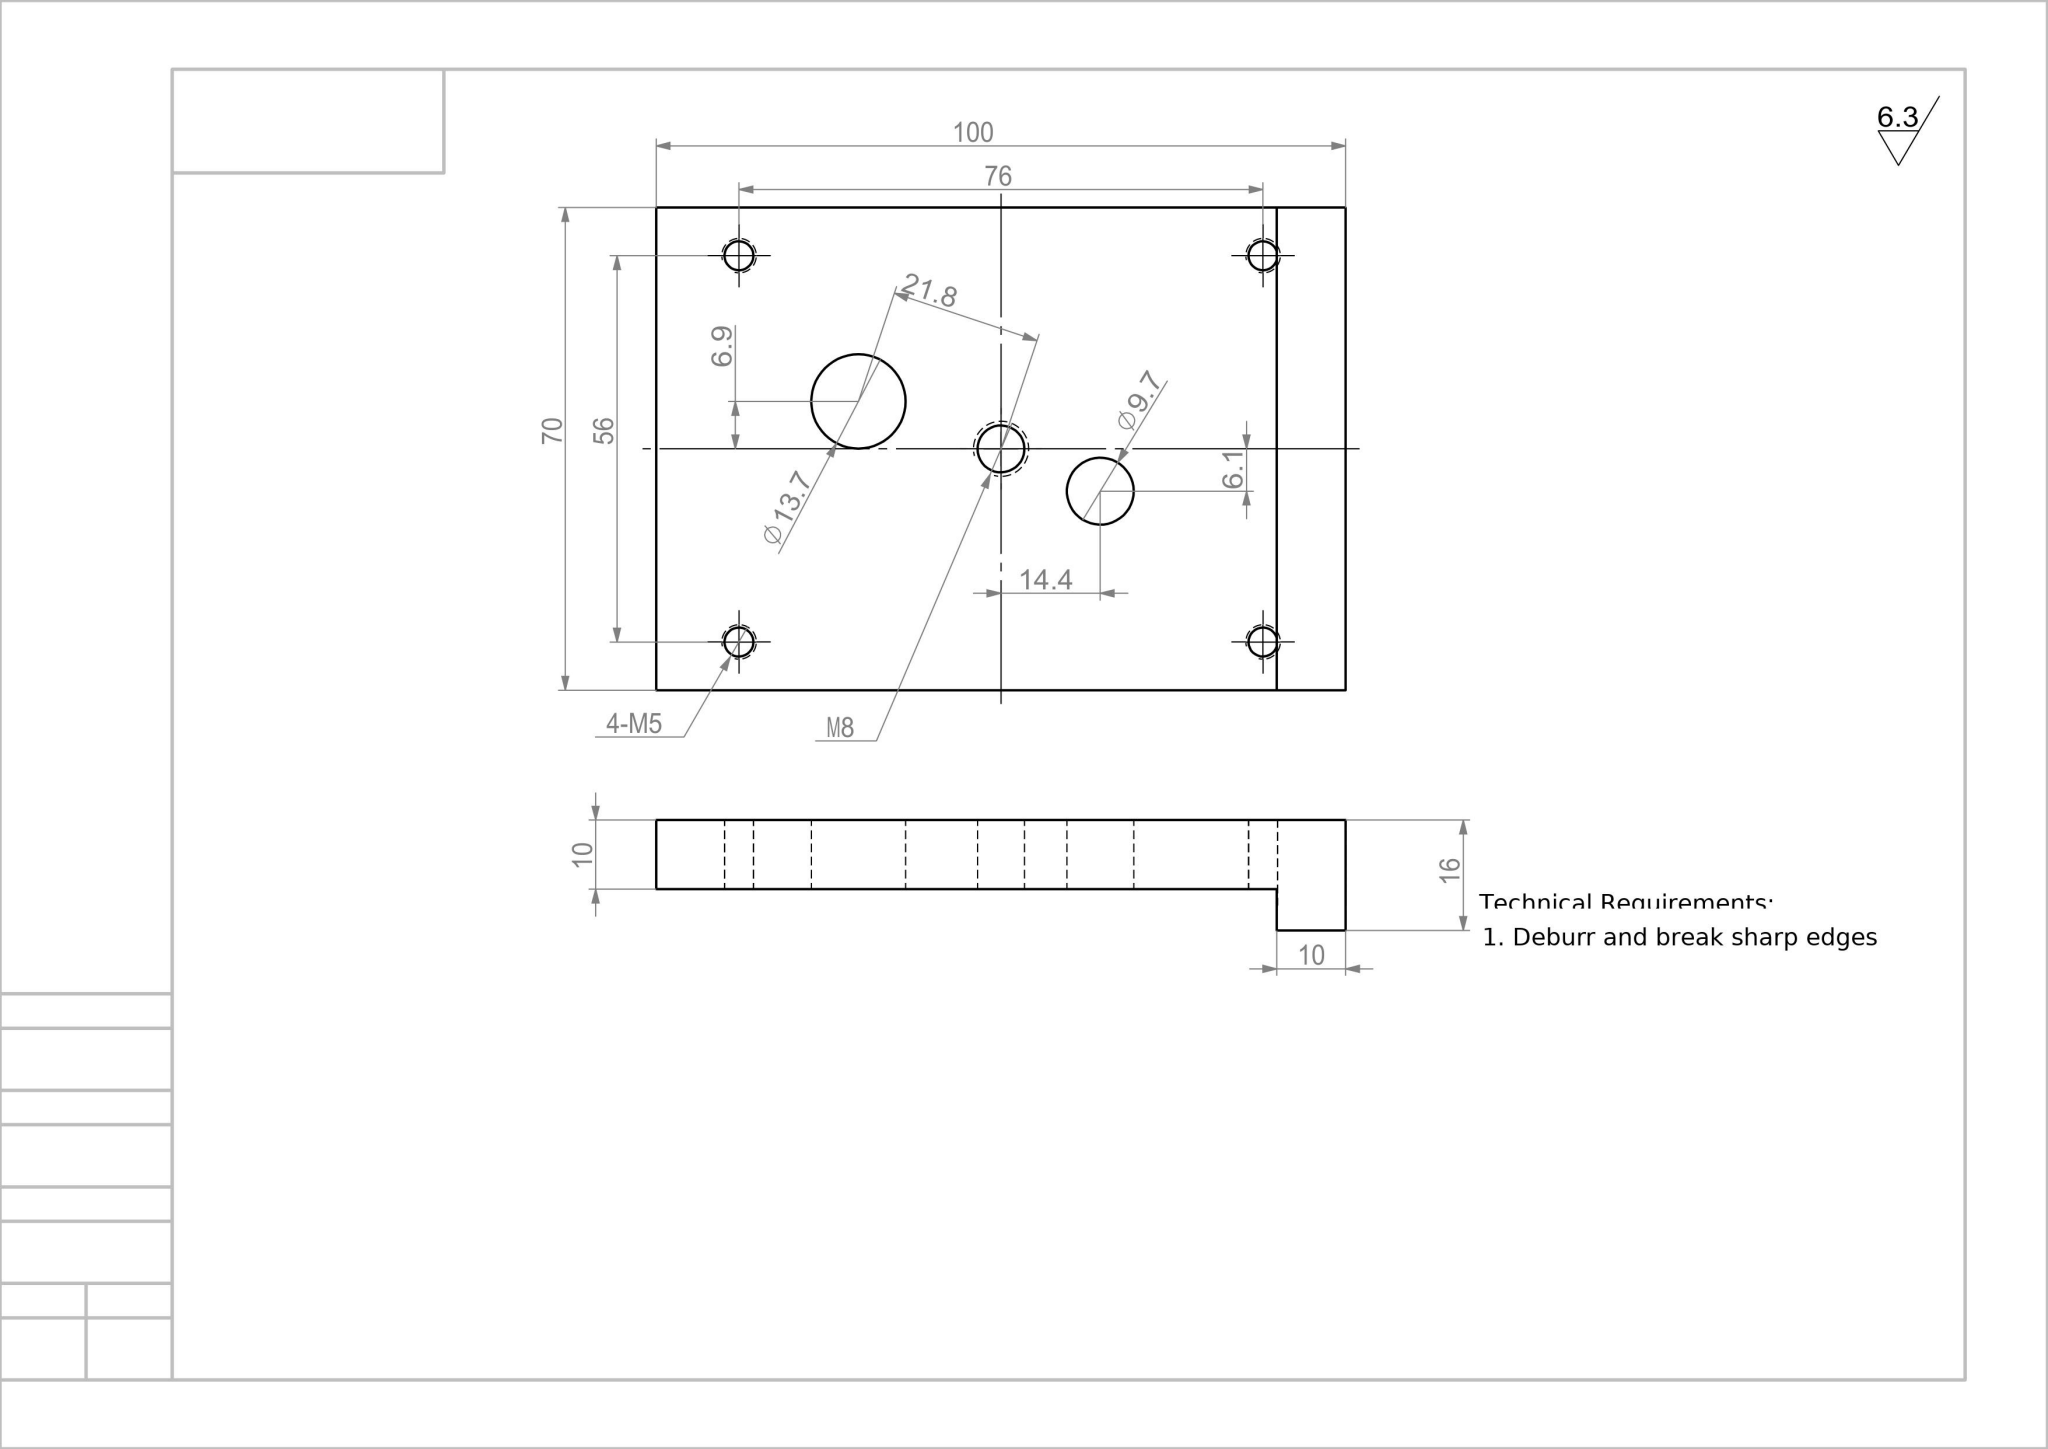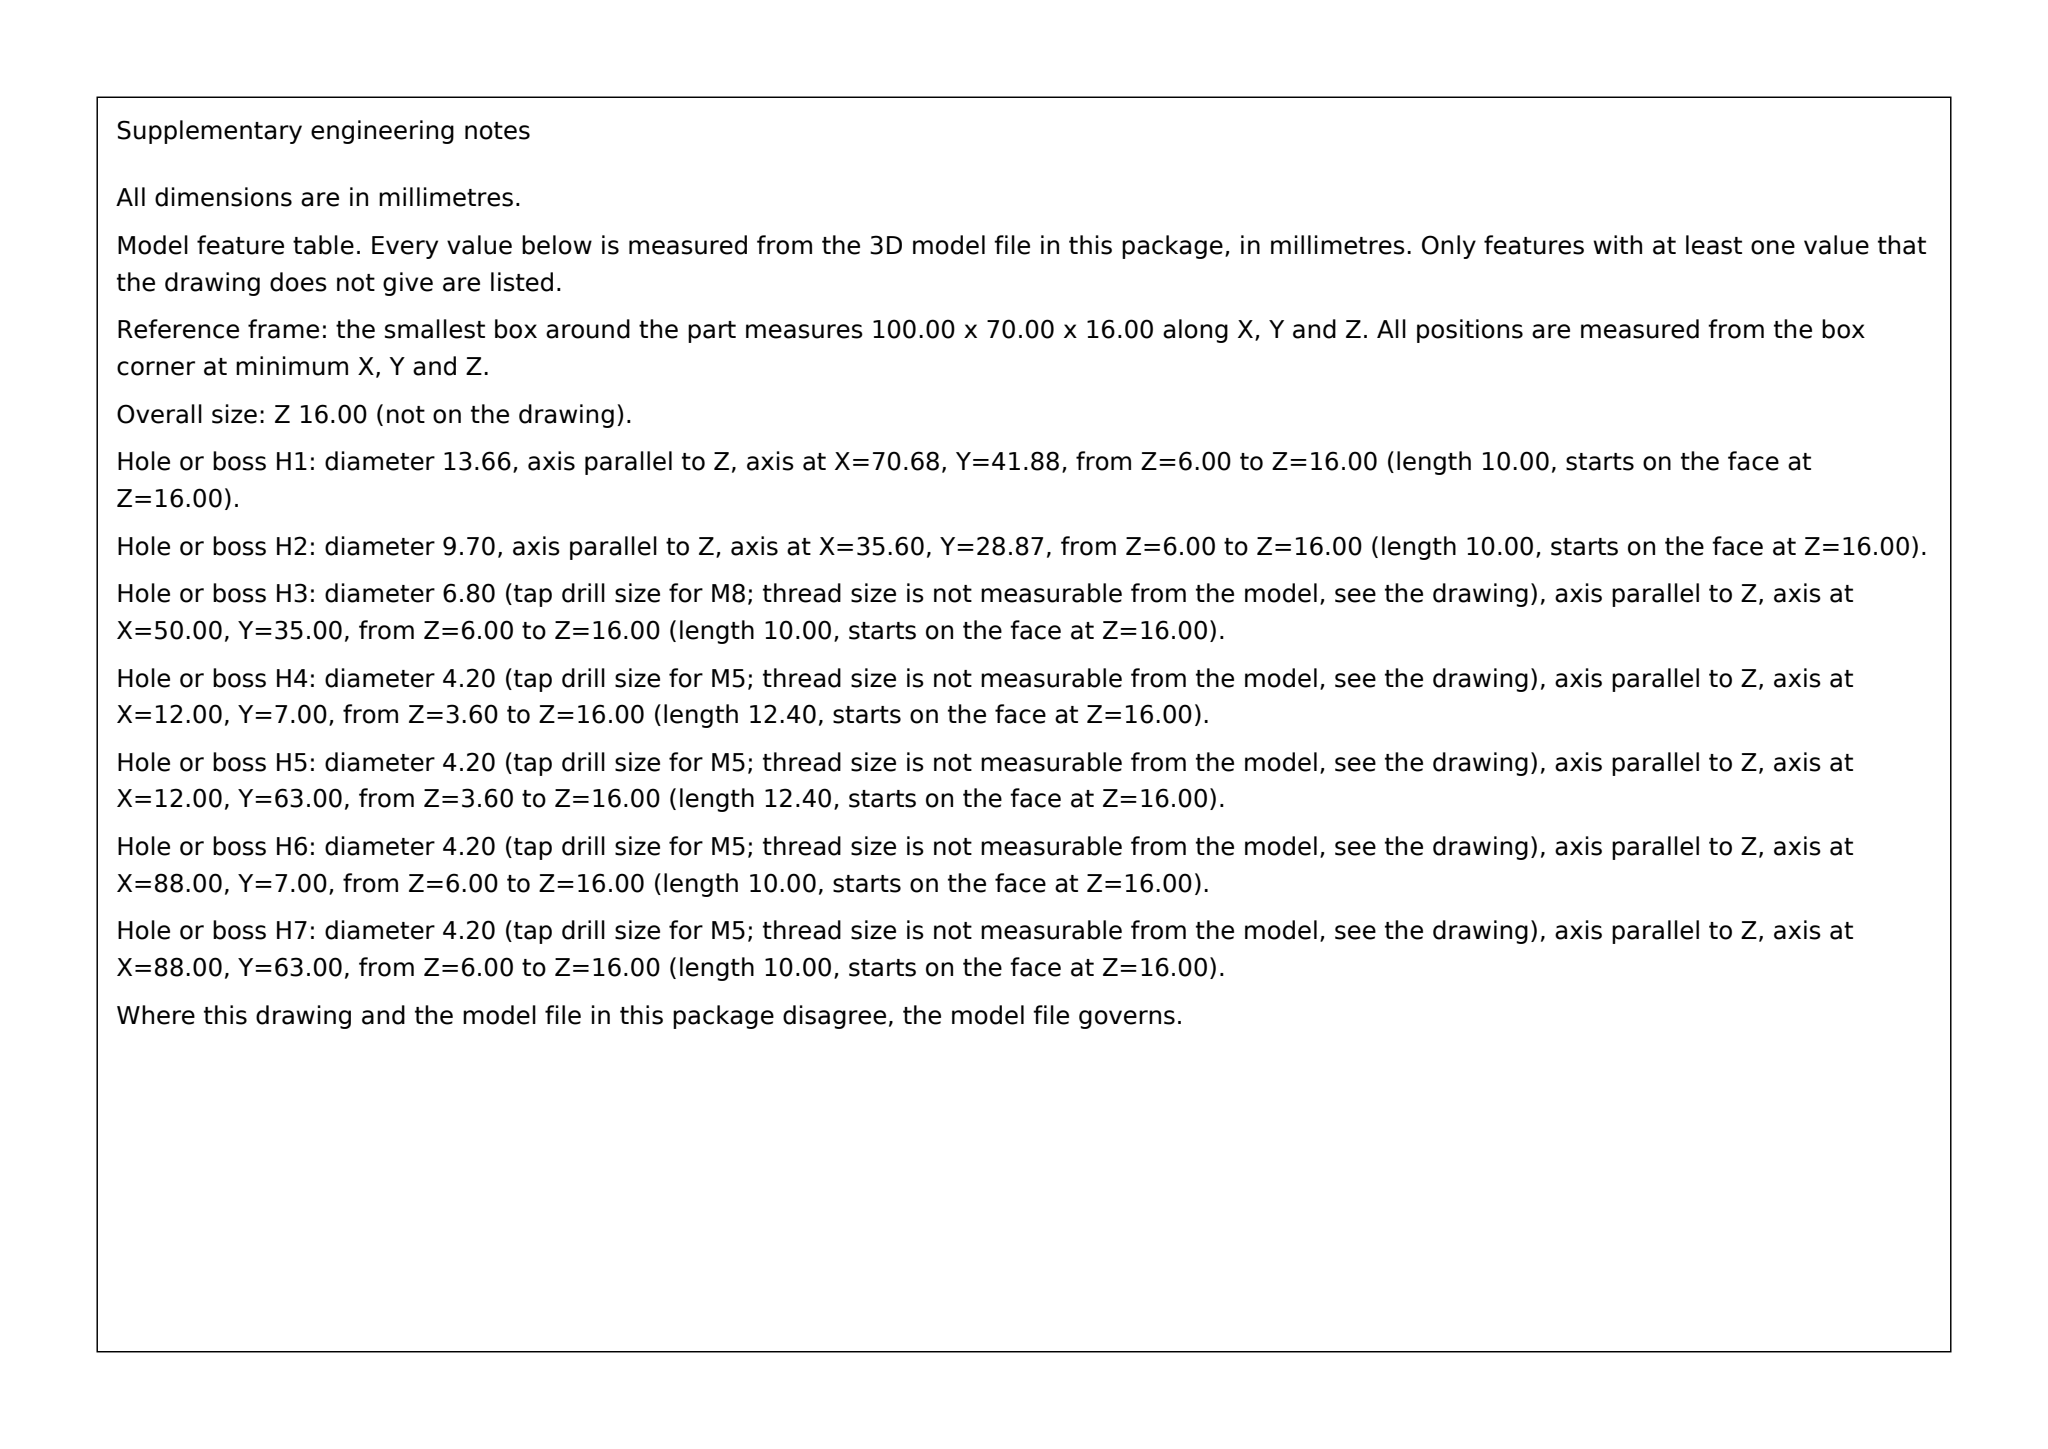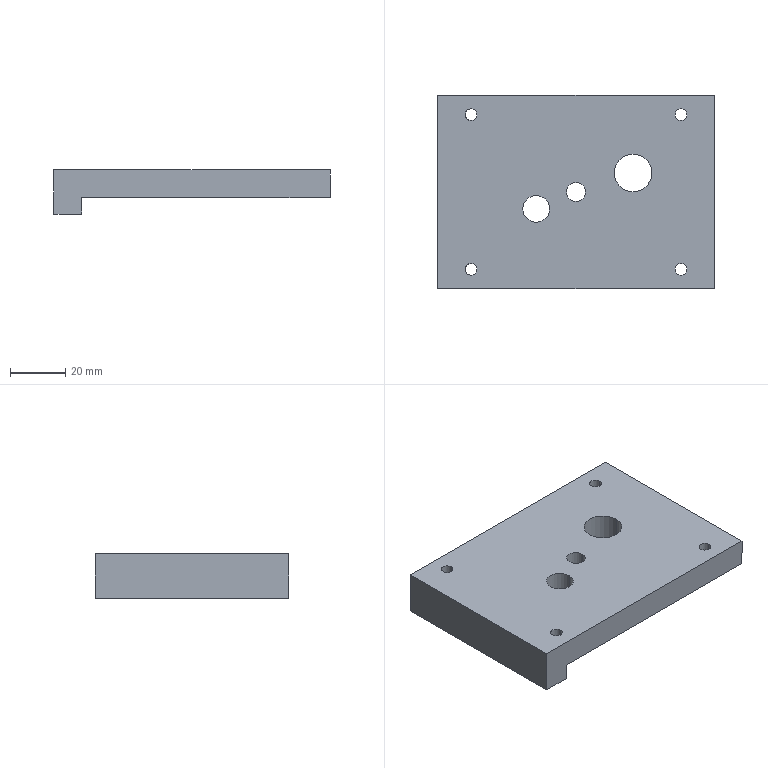Part | SolidWorks | mm | 1 solid | 24 faces | box 100 x 70 x 16 mm | volume 71076 mm3 | cylinder 14 | plane 8 | cone 2 | commonest cylinder face diameters 4.2 x8 13.667 x2 9.702 x2 6.8 x2
build123d program:
from build123d import *

# Parameters (mm, degrees)
SKETCH1_W                  = 100
SKETCH1_H                  = 70
BOSS_EXTRUDE1_DEPTH        = 16
M8_TAPPED_HOLE1_D          = 6.8
M8_TAPPED_HOLE1_DEPTH      = 19.75
M8_TAPPED_HOLE1_TIP        = 2.043
SKETCH3_W                  = 92.5
SKETCH3_H                  = 6
CUT_EXTRUDE1_DEPTH         = 88.499
M5_TAPPED_HOLE1_AT_2_COUNT = 2
M5_TAPPED_HOLE1_AT_2_PITCH = 56
SKETCH5_R                  = 6.834
SKETCH5_R_2                = 4.851
CUT_EXTRUDE2_DEPTH         = 80


with BuildPart() as part:
    # Sketch1 → Boss-Extrude1 (new body)
    with BuildSketch(Plane.XY):
        Rectangle(SKETCH1_W, SKETCH1_H)
    extrude(amount=BOSS_EXTRUDE1_DEPTH)

    # M8 Tapped Hole1
    with Locations(Plane.XY.offset(16)):
        with Locations((0, 0)):
            Hole(M8_TAPPED_HOLE1_D / 2, depth=M8_TAPPED_HOLE1_DEPTH)
            with Locations((0, 0, -(M8_TAPPED_HOLE1_DEPTH + M8_TAPPED_HOLE1_TIP / 2))):  # 118° drill point
                Cone(0, M8_TAPPED_HOLE1_D / 2, M8_TAPPED_HOLE1_TIP, mode=Mode.SUBTRACT)

    # Sketch3 → Cut-Extrude1 (cut, through all)
    with BuildSketch(Plane(origin=(0, 35, 0), x_dir=(1, 0, 0), z_dir=(0, 1, 0))):
        with Locations((6.25, -3)):
            Rectangle(SKETCH3_W, SKETCH3_H)
    extrude(amount=-CUT_EXTRUDE1_DEPTH, mode=Mode.SUBTRACT)

    # Sketch4 → M5 Tapped Hole1 (revolve, cut)
    with BuildSketch(Plane(origin=(-38, 28, 16), x_dir=(0, -1, 0), z_dir=(1, 0, 0))):
        Polygon((0, 0), (0, 13.662), (2.1, 12.4), (2.1, 0), align=None)
    m5_tapped_hole1 = revolve(axis=Axis((-38, 28, 22.35), (0, 0, -1)), mode=Mode.SUBTRACT)

    # M5 Tapped Hole1 at 2: M5 Tapped Hole1 ×2
    with Locations(*[(0, -i * M5_TAPPED_HOLE1_AT_2_PITCH, 0) for i in range(1, M5_TAPPED_HOLE1_AT_2_COUNT)]):
        add(m5_tapped_hole1, mode=Mode.SUBTRACT)

    # Mirror1: M5 Tapped Hole1 across plane
    add(m5_tapped_hole1.mirror(Plane(origin=(0, 0, 0), x_dir=(0, 0, 1), z_dir=(1, 0, 0))), mode=Mode.SUBTRACT)

    # Mirror1 copy 1 sketch → Mirror1 copy 1 (revolve, cut)
    with BuildSketch(Plane(origin=(38, -28, 16), x_dir=(0, -1, 0), z_dir=(-1, 0, 0))):
        Polygon((0, 0), (0, -13.662), (2.1, -12.4), (2.1, 0), align=None)
    revolve(axis=Axis((38, -28, 22.35), (0, 0, 1)), mode=Mode.SUBTRACT)

    # Sketch5 → Cut-Extrude2 (cut)
    with BuildSketch(Plane(origin=(0, 0, 6), x_dir=(-1, 0, 0), z_dir=(0, 0, -1))):
        with Locations((-20.676, 6.881)):
            Circle(SKETCH5_R)
        with Locations((14.404, -6.129)):
            Circle(SKETCH5_R_2)
    extrude(amount=-CUT_EXTRUDE2_DEPTH, mode=Mode.SUBTRACT)


solid = part.part